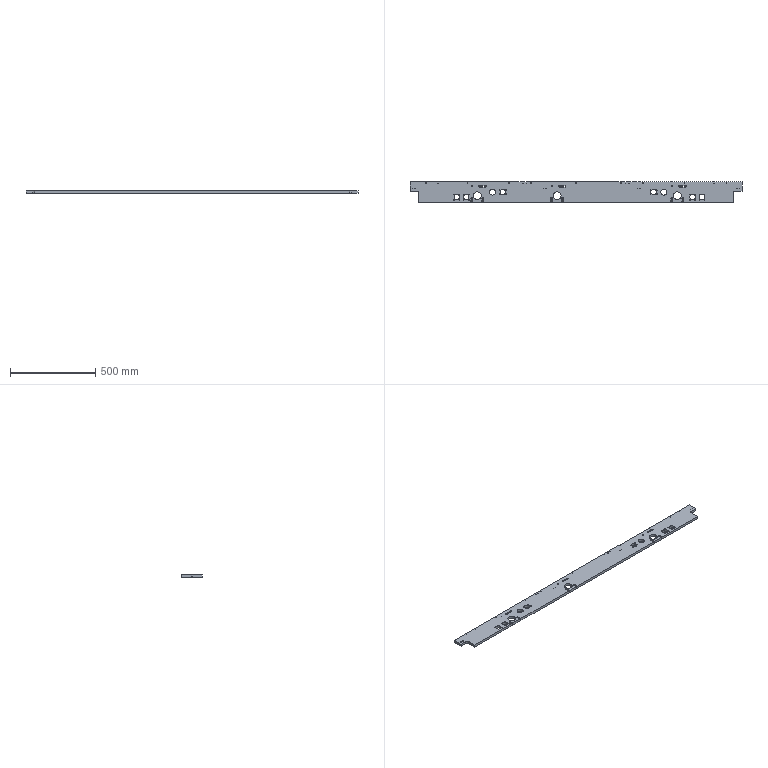Component | SolidWorks | SL010-RightStreamline-1-1_SL010-LXFB-010203-01-1 | 1 solid | 263 faces | volume 3176843 mm3 | cylinder 208 | plane 37 | cone 18 | commonest cylinder face diameters 4.2 x50 2.5 x34 10 x33 5.5 x33 3.3 x18 5 x16 32 x12 46 x6 | material Aluminum-6061